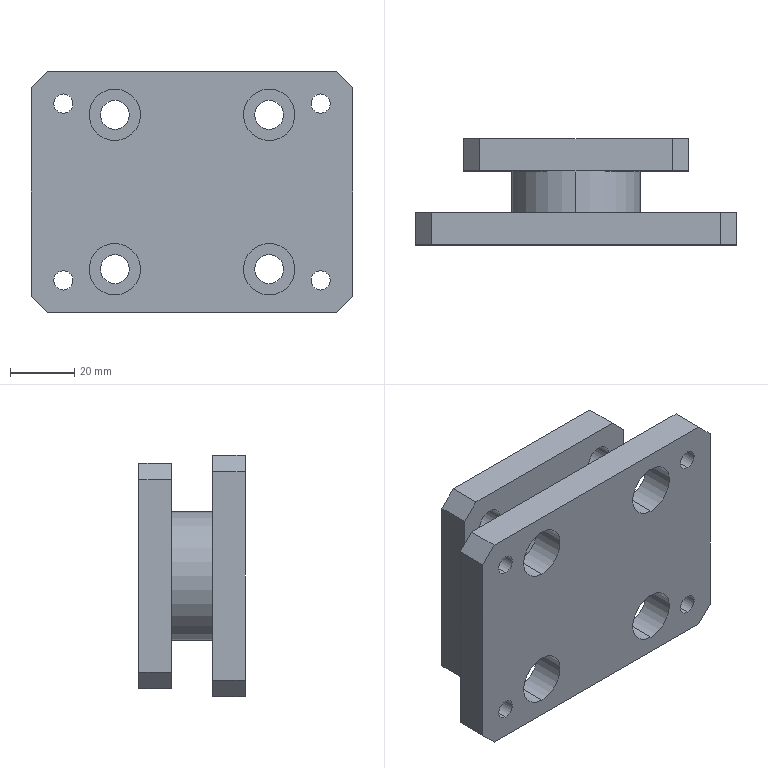Component | SolidWorks | RisingBeltCylinderSeat-1 | 1 solid | 58 faces | box 100 x 33 x 75 mm | volume 126911 mm3 | cylinder 34 | plane 24 | commonest cylinder face diameters 9 x16 16 x8 6 x8 40 x2
build123d program:
from build123d import *

# Parameters (mm, degrees)
SKETCH1_W                                           = 100
SKETCH1_H                                           = 75
BOSS_EXTRUDE1_DEPTH                                 = 10
SKETCH2_R                                           = 20
BOSS_EXTRUDE2_DEPTH                                 = 13
SKETCH3_W                                           = 70
SKETCH3_H                                           = 70
BOSS_EXTRUDE3_DEPTH                                 = 10
CYLINDRICAL_COUNTERSUNK_HOLE_FOR_M5_HEX_D           = 6
CYLINDRICAL_COUNTERSUNK_HOLE_FOR_M5_HEX_CBORE_D     = 9
CYLINDRICAL_COUNTERSUNK_HOLE_FOR_M5_HEX_CBORE_DEPTH = 5
CIRPATTERN1_COUNT                                   = 4
SKETCH10_R                                          = 8
CUT_EXTRUDE1_DEPTH                                  = 67.598
CIRPATTERN2_COUNT                                   = 4
CHAMFER1_SIZE                                       = 5
CHAMFER2_SIZE                                       = 5


with BuildPart() as part:
    # Sketch1 → Boss-Extrude1 (new body)
    with BuildSketch(Plane(origin=(0, 0, 0), x_dir=(1, 0, 0), z_dir=(0, 1, 0))):
        Rectangle(SKETCH1_W, SKETCH1_H)
    extrude(amount=BOSS_EXTRUDE1_DEPTH)

    # Sketch2 → Boss-Extrude2 (add)
    with BuildSketch(Plane(origin=(0, 10, 0), x_dir=(1, 0, 0), z_dir=(0, 1, 0))):
        with Locations(Location((0, 0, 0), (0, 0, 90))):
            Circle(SKETCH2_R)
    extrude(amount=BOSS_EXTRUDE2_DEPTH)

    # Sketch3 → Boss-Extrude3 (add)
    with BuildSketch(Plane(origin=(0, 23, 0), x_dir=(1, 0, 0), z_dir=(0, 1, 0))):
        Rectangle(SKETCH3_W, SKETCH3_H)
    extrude(amount=BOSS_EXTRUDE3_DEPTH)

    # Sketch7 → 9.0 _9_ Diameter Hole1 (revolve, cut)
    with BuildSketch(Plane(origin=(-24, 23, -24), x_dir=(0, 0, -1), z_dir=(1, 0, 0))):
        Polygon((0, 0), (0, 15.104), (4.5, 12.4), (4.5, 0), align=None)
    f_9_0_9_diameter_hole1 = revolve(axis=Axis((-24, 16.65, -24), (0, 1, 0)), mode=Mode.SUBTRACT)

    # Cylindrical Countersunk Hole for M5 Hex (through all)
    with Locations(Plane(origin=(0, 10, 0), x_dir=(1, 0, 0), z_dir=(0, 1, 0))):
        with Locations((-40, 27.5), (40, 27.5), (40, -27.5), (-40, -27.5)):
            CounterBoreHole(CYLINDRICAL_COUNTERSUNK_HOLE_FOR_M5_HEX_D / 2, CYLINDRICAL_COUNTERSUNK_HOLE_FOR_M5_HEX_CBORE_D / 2, CYLINDRICAL_COUNTERSUNK_HOLE_FOR_M5_HEX_CBORE_DEPTH)

    # CirPattern1: 9.0 _9_ Diameter Hole1 ×4 about axis
    cirpattern1_axis = Axis((0, 0, 0), (0, 1, 0))
    for i in range(1, CIRPATTERN1_COUNT):
        add(f_9_0_9_diameter_hole1.rotate(cirpattern1_axis, i * 360 / CIRPATTERN1_COUNT), mode=Mode.SUBTRACT)

    # Sketch10 → Cut-Extrude1 (cut, through all)
    with BuildSketch(Plane(origin=(0, 10, 0), x_dir=(1, 0, 0), z_dir=(0, 1, 0))):
        with Locations(Location((-24, 24, 0), (0, 0, 270))):
            Circle(SKETCH10_R)
    cut_extrude1 = extrude(amount=-CUT_EXTRUDE1_DEPTH, mode=Mode.SUBTRACT)

    # CirPattern2: Cut-Extrude1 ×4 about axis
    cirpattern2_axis = Axis((0, 0, 0), (0, 1, 0))
    for i in range(1, CIRPATTERN2_COUNT):
        add(cut_extrude1.rotate(cirpattern2_axis, i * 360 / CIRPATTERN2_COUNT), mode=Mode.SUBTRACT)

    # Chamfer1
    chamfer1_edges = [part.edges().sort_by_distance(p)[0] for p in [
        (35, 28, 35),
        (35, 28, -35),
        (-35, 28, -35),
        (-35, 28, 35),
    ]]
    chamfer(chamfer1_edges, length=CHAMFER1_SIZE)

    # Chamfer2
    chamfer2_edges = [part.edges().sort_by_distance(p)[0] for p in [
        (-50, 5, -37.5),
        (50, 5, -37.5),
        (50, 5, 37.5),
        (-50, 5, 37.5),
    ]]
    chamfer(chamfer2_edges, length=CHAMFER2_SIZE)


solid = part.part

# Placed as in the assembly
solid = solid.moved(Location((-29.507, -289.411, 430.5), (0, 0, 0)))